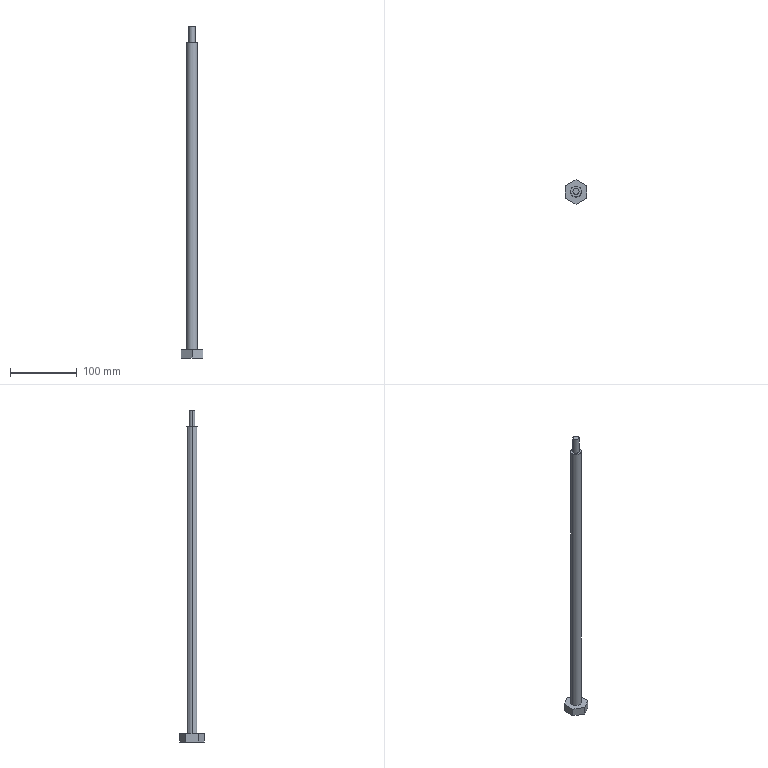Component | SolidWorks | HangerRod-1 | 1 solid | 14 faces | box 32 x 36.95 x 497 mm | volume 104721 mm3 | plane 10 | cylinder 4 | commonest cylinder face diameters 9 x2 16 x2
build123d program:
from build123d import *

# Parameters (mm, degrees)
BOSS_EXTRUDE1_DEPTH = 12
SKETCH2_R           = 8
BOSS_EXTRUDE2_DEPTH = 485
CHAMFER1_SIZE       = 1
SKETCH1_R           = 10
SKETCH1_R_2         = 4.5
CUT_EXTRUDE1_DEPTH  = 25


with BuildPart() as part:
    # Sketch1_2 → Boss-Extrude1 (new body)
    with BuildSketch(Plane.XY):
        Polygon((0, 18.475), (-16, 9.238), (-16, -9.238), (0, -18.475), (16, -9.238), (16, 9.238), align=None)
    extrude(amount=BOSS_EXTRUDE1_DEPTH)

    # Sketch2 → Boss-Extrude2 (add)
    with BuildSketch(Plane.XY.offset(12)):
        Circle(SKETCH2_R)
    extrude(amount=BOSS_EXTRUDE2_DEPTH)

    # Chamfer1
    chamfer1_edges = [part.edges().sort_by_distance(p)[0] for p in [
        (-8, 0, 497),
    ]]
    chamfer(chamfer1_edges, length=CHAMFER1_SIZE)

    # Sketch1 → Cut-Extrude1 (cut)
    with BuildSketch(Plane.XY.offset(497)):
        Circle(SKETCH1_R)
        Circle(SKETCH1_R_2, mode=Mode.SUBTRACT)
    extrude(amount=-CUT_EXTRUDE1_DEPTH, mode=Mode.SUBTRACT)


solid = part.part

# Placed as in the assembly
solid = solid.moved(Location((-917, 348, -612), (0, 0, 0)))
STEP:
#1=COLOUR_RGB('',0.7922,0.8196,0.9333);
#2=FILL_AREA_STYLE_COLOUR('',#1);
#3=FILL_AREA_STYLE('',(#2));
#4=SURFACE_STYLE_FILL_AREA(#3);
#5=SURFACE_SIDE_STYLE('',(#4));
#6=SURFACE_STYLE_USAGE(.BOTH.,#5);
#7=PRESENTATION_STYLE_ASSIGNMENT((#6));
#8=CARTESIAN_POINT('',(-35.925,13.701,-5.512));
#9=VERTEX_POINT('',#8);
#10=CARTESIAN_POINT('',(-36.28,13.701,-5.512));
#11=VERTEX_POINT('',#10);
#12=CARTESIAN_POINT('',(-36.102,13.701,-5.512));
#13=DIRECTION('',(0.,0.,1.));
#14=DIRECTION('',(1.,0.,0.));
#15=AXIS2_PLACEMENT_3D('',#12,#13,#14);
#16=CIRCLE('',#15,0.1772);
#17=EDGE_CURVE('',#9,#11,#16,.T.);
#18=ORIENTED_EDGE('',*,*,#17,.T.);
#19=CARTESIAN_POINT('',(-36.28,13.701,-4.528));
#20=VERTEX_POINT('',#19);
#21=CARTESIAN_POINT('',(-36.28,13.701,-5.512));
#22=DIRECTION('',(0.,0.,1.));
#23=VECTOR('',#22,39.37);
#24=LINE('',#21,#23);
#25=EDGE_CURVE('',#11,#20,#24,.T.);
#26=ORIENTED_EDGE('',*,*,#25,.T.);
#27=CARTESIAN_POINT('',(-35.925,13.701,-4.528));
#28=VERTEX_POINT('',#27);
#29=CARTESIAN_POINT('',(-36.102,13.701,-4.528));
#30=DIRECTION('',(0.,0.,1.));
#31=DIRECTION('',(1.,0.,0.));
#32=AXIS2_PLACEMENT_3D('',#29,#30,#31);
#33=CIRCLE('',#32,0.1772);
#34=EDGE_CURVE('',#28,#20,#33,.T.);
#35=ORIENTED_EDGE('',*,*,#34,.F.);
#36=CARTESIAN_POINT('',(-35.925,13.701,-5.512));
#37=DIRECTION('',(0.,0.,1.));
#38=VECTOR('',#37,39.37);
#39=LINE('',#36,#38);
#40=EDGE_CURVE('',#9,#28,#39,.T.);
#41=ORIENTED_EDGE('',*,*,#40,.F.);
#42=EDGE_LOOP('',(#18,#26,#35,#41));
#43=FACE_OUTER_BOUND('',#42,.T.);
#44=CARTESIAN_POINT('',(-36.102,13.701,-5.512));
#45=DIRECTION('',(0.,0.,1.));
#46=DIRECTION('',(1.,0.,0.));
#47=AXIS2_PLACEMENT_3D('',#44,#45,#46);
#48=CYLINDRICAL_SURFACE('',#47,0.1772);
#49=ADVANCED_FACE('',(#43),#48,.T.);
#50=CARTESIAN_POINT('',(-35.787,13.701,-5.512));
#51=VERTEX_POINT('',#50);
#52=CARTESIAN_POINT('',(-36.417,13.701,-5.512));
#53=VERTEX_POINT('',#52);
#54=CARTESIAN_POINT('',(-36.102,13.701,-5.512));
#55=DIRECTION('',(0.,0.,1.));
#56=DIRECTION('',(1.,0.,0.));
#57=AXIS2_PLACEMENT_3D('',#54,#55,#56);
#58=CIRCLE('',#57,0.315);
#59=EDGE_CURVE('',#51,#53,#58,.T.);
#60=ORIENTED_EDGE('',*,*,#59,.F.);
#61=CARTESIAN_POINT('',(-35.787,13.701,-23.622));
#62=VERTEX_POINT('',#61);
#63=CARTESIAN_POINT('',(-35.787,13.701,-4.528));
#64=DIRECTION('',(0.,0.,-1.));
#65=VECTOR('',#64,39.37);
#66=LINE('',#63,#65);
#67=EDGE_CURVE('',#51,#62,#66,.T.);
#68=ORIENTED_EDGE('',*,*,#67,.T.);
#69=CARTESIAN_POINT('',(-36.417,13.701,-23.622));
#70=VERTEX_POINT('',#69);
#71=CARTESIAN_POINT('',(-36.102,13.701,-23.622));
#72=DIRECTION('',(0.,0.,1.));
#73=DIRECTION('',(1.,0.,0.));
#74=AXIS2_PLACEMENT_3D('',#71,#72,#73);
#75=CIRCLE('',#74,0.315);
#76=EDGE_CURVE('',#62,#70,#75,.T.);
#77=ORIENTED_EDGE('',*,*,#76,.T.);
#78=CARTESIAN_POINT('',(-36.417,13.701,-4.528));
#79=DIRECTION('',(0.,0.,-1.));
#80=VECTOR('',#79,39.37);
#81=LINE('',#78,#80);
#82=EDGE_CURVE('',#53,#70,#81,.T.);
#83=ORIENTED_EDGE('',*,*,#82,.F.);
#84=EDGE_LOOP('',(#60,#68,#77,#83));
#85=FACE_OUTER_BOUND('',#84,.T.);
#86=CARTESIAN_POINT('',(-36.102,13.701,-4.528));
#87=DIRECTION('',(0.,0.,-1.));
#88=DIRECTION('',(-1.,0.,0.));
#89=AXIS2_PLACEMENT_3D('',#86,#87,#88);
#90=CYLINDRICAL_SURFACE('',#89,0.315);
#91=ADVANCED_FACE('',(#85),#90,.T.);
#92=ORIENTED_EDGE('',*,*,#67,.F.);
#93=CARTESIAN_POINT('',(-36.102,13.701,-5.512));
#94=DIRECTION('',(0.,0.,1.));
#95=DIRECTION('',(1.,0.,0.));
#96=AXIS2_PLACEMENT_3D('',#93,#94,#95);
#97=CIRCLE('',#96,0.315);
#98=EDGE_CURVE('',#53,#51,#97,.T.);
#99=ORIENTED_EDGE('',*,*,#98,.F.);
#100=ORIENTED_EDGE('',*,*,#82,.T.);
#101=CARTESIAN_POINT('',(-36.102,13.701,-23.622));
#102=DIRECTION('',(0.,0.,1.));
#103=DIRECTION('',(1.,0.,0.));
#104=AXIS2_PLACEMENT_3D('',#101,#102,#103);
#105=CIRCLE('',#104,0.315);
#106=EDGE_CURVE('',#70,#62,#105,.T.);
#107=ORIENTED_EDGE('',*,*,#106,.T.);
#108=EDGE_LOOP('',(#92,#99,#100,#107));
#109=FACE_OUTER_BOUND('',#108,.T.);
#110=CARTESIAN_POINT('',(-36.102,13.701,-4.528));
#111=DIRECTION('',(0.,0.,-1.));
#112=DIRECTION('',(-1.,0.,0.));
#113=AXIS2_PLACEMENT_3D('',#110,#111,#112);
#114=CYLINDRICAL_SURFACE('',#113,0.315);
#115=ADVANCED_FACE('',(#109),#114,.T.);
#116=CARTESIAN_POINT('',(-35.472,14.064,-23.622));
#117=VERTEX_POINT('',#116);
#118=CARTESIAN_POINT('',(-36.102,14.428,-23.622));
#119=VERTEX_POINT('',#118);
#120=CARTESIAN_POINT('',(-35.472,14.064,-23.622));
#121=DIRECTION('',(-0.866,0.5,0.));
#122=VECTOR('',#121,39.37);
#123=LINE('',#120,#122);
#124=EDGE_CURVE('',#117,#119,#123,.T.);
#125=ORIENTED_EDGE('',*,*,#124,.T.);
#126=CARTESIAN_POINT('',(-36.732,14.064,-23.622));
#127=VERTEX_POINT('',#126);
#128=CARTESIAN_POINT('',(-36.102,14.428,-23.622));
#129=DIRECTION('',(-0.866,-0.5,0.));
#130=VECTOR('',#129,39.37);
#131=LINE('',#128,#130);
#132=EDGE_CURVE('',#119,#127,#131,.T.);
#133=ORIENTED_EDGE('',*,*,#132,.T.);
#134=CARTESIAN_POINT('',(-36.732,13.337,-23.622));
#135=VERTEX_POINT('',#134);
#136=CARTESIAN_POINT('',(-36.732,14.064,-23.622));
#137=DIRECTION('',(0.,-1.,0.));
#138=VECTOR('',#137,39.37);
#139=LINE('',#136,#138);
#140=EDGE_CURVE('',#127,#135,#139,.T.);
#141=ORIENTED_EDGE('',*,*,#140,.T.);
#142=CARTESIAN_POINT('',(-36.102,12.973,-23.622));
#143=VERTEX_POINT('',#142);
#144=CARTESIAN_POINT('',(-36.732,13.337,-23.622));
#145=DIRECTION('',(0.866,-0.5,0.));
#146=VECTOR('',#145,39.37);
#147=LINE('',#144,#146);
#148=EDGE_CURVE('',#135,#143,#147,.T.);
#149=ORIENTED_EDGE('',*,*,#148,.T.);
#150=CARTESIAN_POINT('',(-35.472,13.337,-23.622));
#151=VERTEX_POINT('',#150);
#152=CARTESIAN_POINT('',(-36.102,12.973,-23.622));
#153=DIRECTION('',(0.866,0.5,0.));
#154=VECTOR('',#153,39.37);
#155=LINE('',#152,#154);
#156=EDGE_CURVE('',#143,#151,#155,.T.);
#157=ORIENTED_EDGE('',*,*,#156,.T.);
#158=CARTESIAN_POINT('',(-35.472,13.337,-23.622));
#159=DIRECTION('',(-0.,1.,0.));
#160=VECTOR('',#159,39.37);
#161=LINE('',#158,#160);
#162=EDGE_CURVE('',#151,#117,#161,.T.);
#163=ORIENTED_EDGE('',*,*,#162,.T.);
#164=EDGE_LOOP('',(#125,#133,#141,#149,#157,#163));
#165=FACE_OUTER_BOUND('',#164,.T.);
#166=ORIENTED_EDGE('',*,*,#106,.F.);
#167=ORIENTED_EDGE('',*,*,#76,.F.);
#168=EDGE_LOOP('',(#166,#167));
#169=FACE_BOUND('',#168,.T.);
#170=CARTESIAN_POINT('',(-36.102,13.701,-23.622));
#171=DIRECTION('',(0.,0.,1.));
#172=DIRECTION('',(1.,0.,0.));
#173=AXIS2_PLACEMENT_3D('',#170,#171,#172);
#174=PLANE('',#173);
#175=ADVANCED_FACE('',(#165,#169),#174,.T.);
#176=CARTESIAN_POINT('',(-35.472,14.064,-24.094));
#177=VERTEX_POINT('',#176);
#178=CARTESIAN_POINT('',(-36.102,14.428,-24.094));
#179=VERTEX_POINT('',#178);
#180=CARTESIAN_POINT('',(-35.472,14.064,-24.094));
#181=DIRECTION('',(-0.866,0.5,0.));
#182=VECTOR('',#181,39.37);
#183=LINE('',#180,#182);
#184=EDGE_CURVE('',#177,#179,#183,.T.);
#185=ORIENTED_EDGE('',*,*,#184,.T.);
#186=CARTESIAN_POINT('',(-36.102,14.428,-23.622));
#187=DIRECTION('',(0.,0.,-1.));
#188=VECTOR('',#187,39.37);
#189=LINE('',#186,#188);
#190=EDGE_CURVE('',#119,#179,#189,.T.);
#191=ORIENTED_EDGE('',*,*,#190,.F.);
#192=ORIENTED_EDGE('',*,*,#124,.F.);
#193=CARTESIAN_POINT('',(-35.472,14.064,-23.622));
#194=DIRECTION('',(0.,0.,-1.));
#195=VECTOR('',#194,39.37);
#196=LINE('',#193,#195);
#197=EDGE_CURVE('',#117,#177,#196,.T.);
#198=ORIENTED_EDGE('',*,*,#197,.T.);
#199=EDGE_LOOP('',(#185,#191,#192,#198));
#200=FACE_OUTER_BOUND('',#199,.T.);
#201=CARTESIAN_POINT('',(-35.472,14.064,-23.622));
#202=DIRECTION('',(-0.5,-0.866,0.));
#203=DIRECTION('',(0.866,-0.5,0.));
#204=AXIS2_PLACEMENT_3D('',#201,#202,#203);
#205=PLANE('',#204);
#206=ADVANCED_FACE('',(#200),#205,.F.);
#207=CARTESIAN_POINT('',(-36.732,14.064,-24.094));
#208=VERTEX_POINT('',#207);
#209=CARTESIAN_POINT('',(-36.102,14.428,-24.094));
#210=DIRECTION('',(-0.866,-0.5,0.));
#211=VECTOR('',#210,39.37);
#212=LINE('',#209,#211);
#213=EDGE_CURVE('',#179,#208,#212,.T.);
#214=ORIENTED_EDGE('',*,*,#213,.T.);
#215=CARTESIAN_POINT('',(-36.732,14.064,-23.622));
#216=DIRECTION('',(0.,0.,-1.));
#217=VECTOR('',#216,39.37);
#218=LINE('',#215,#217);
#219=EDGE_CURVE('',#127,#208,#218,.T.);
#220=ORIENTED_EDGE('',*,*,#219,.F.);
#221=ORIENTED_EDGE('',*,*,#132,.F.);
#222=ORIENTED_EDGE('',*,*,#190,.T.);
#223=EDGE_LOOP('',(#214,#220,#221,#222));
#224=FACE_OUTER_BOUND('',#223,.T.);
#225=CARTESIAN_POINT('',(-36.102,14.428,-23.622));
#226=DIRECTION('',(0.5,-0.866,0.));
#227=DIRECTION('',(0.866,0.5,0.));
#228=AXIS2_PLACEMENT_3D('',#225,#226,#227);
#229=PLANE('',#228);
#230=ADVANCED_FACE('',(#224),#229,.F.);
#231=CARTESIAN_POINT('',(-36.732,13.337,-24.094));
#232=VERTEX_POINT('',#231);
#233=CARTESIAN_POINT('',(-36.732,14.064,-24.094));
#234=DIRECTION('',(0.,-1.,0.));
#235=VECTOR('',#234,39.37);
#236=LINE('',#233,#235);
#237=EDGE_CURVE('',#208,#232,#236,.T.);
#238=ORIENTED_EDGE('',*,*,#237,.T.);
#239=CARTESIAN_POINT('',(-36.732,13.337,-23.622));
#240=DIRECTION('',(0.,0.,-1.));
#241=VECTOR('',#240,39.37);
#242=LINE('',#239,#241);
#243=EDGE_CURVE('',#135,#232,#242,.T.);
#244=ORIENTED_EDGE('',*,*,#243,.F.);
#245=ORIENTED_EDGE('',*,*,#140,.F.);
#246=ORIENTED_EDGE('',*,*,#219,.T.);
#247=EDGE_LOOP('',(#238,#244,#245,#246));
#248=FACE_OUTER_BOUND('',#247,.T.);
#249=CARTESIAN_POINT('',(-36.732,14.064,-23.622));
#250=DIRECTION('',(1.,0.,0.));
#251=DIRECTION('',(-0.,1.,0.));
#252=AXIS2_PLACEMENT_3D('',#249,#250,#251);
#253=PLANE('',#252);
#254=ADVANCED_FACE('',(#248),#253,.F.);
#255=CARTESIAN_POINT('',(-36.102,12.973,-24.094));
#256=VERTEX_POINT('',#255);
#257=CARTESIAN_POINT('',(-36.732,13.337,-24.094));
#258=DIRECTION('',(0.866,-0.5,0.));
#259=VECTOR('',#258,39.37);
#260=LINE('',#257,#259);
#261=EDGE_CURVE('',#232,#256,#260,.T.);
#262=ORIENTED_EDGE('',*,*,#261,.T.);
#263=CARTESIAN_POINT('',(-36.102,12.973,-23.622));
#264=DIRECTION('',(0.,0.,-1.));
#265=VECTOR('',#264,39.37);
#266=LINE('',#263,#265);
#267=EDGE_CURVE('',#143,#256,#266,.T.);
#268=ORIENTED_EDGE('',*,*,#267,.F.);
#269=ORIENTED_EDGE('',*,*,#148,.F.);
#270=ORIENTED_EDGE('',*,*,#243,.T.);
#271=EDGE_LOOP('',(#262,#268,#269,#270));
#272=FACE_OUTER_BOUND('',#271,.T.);
#273=CARTESIAN_POINT('',(-36.732,13.337,-23.622));
#274=DIRECTION('',(0.5,0.866,0.));
#275=DIRECTION('',(-0.866,0.5,0.));
#276=AXIS2_PLACEMENT_3D('',#273,#274,#275);
#277=PLANE('',#276);
#278=ADVANCED_FACE('',(#272),#277,.F.);
#279=CARTESIAN_POINT('',(-35.472,13.337,-24.094));
#280=VERTEX_POINT('',#279);
#281=CARTESIAN_POINT('',(-36.102,12.973,-24.094));
#282=DIRECTION('',(0.866,0.5,0.));
#283=VECTOR('',#282,39.37);
#284=LINE('',#281,#283);
#285=EDGE_CURVE('',#256,#280,#284,.T.);
#286=ORIENTED_EDGE('',*,*,#285,.T.);
#287=CARTESIAN_POINT('',(-35.472,13.337,-23.622));
#288=DIRECTION('',(0.,0.,-1.));
#289=VECTOR('',#288,39.37);
#290=LINE('',#287,#289);
#291=EDGE_CURVE('',#151,#280,#290,.T.);
#292=ORIENTED_EDGE('',*,*,#291,.F.);
#293=ORIENTED_EDGE('',*,*,#156,.F.);
#294=ORIENTED_EDGE('',*,*,#267,.T.);
#295=EDGE_LOOP('',(#286,#292,#293,#294));
#296=FACE_OUTER_BOUND('',#295,.T.);
#297=CARTESIAN_POINT('',(-36.102,12.973,-23.622));
#298=DIRECTION('',(-0.5,0.866,0.));
#299=DIRECTION('',(-0.866,-0.5,0.));
#300=AXIS2_PLACEMENT_3D('',#297,#298,#299);
#301=PLANE('',#300);
#302=ADVANCED_FACE('',(#296),#301,.F.);
#303=CARTESIAN_POINT('',(-35.472,13.337,-24.094));
#304=DIRECTION('',(-0.,1.,0.));
#305=VECTOR('',#304,39.37);
#306=LINE('',#303,#305);
#307=EDGE_CURVE('',#280,#177,#306,.T.);
#308=ORIENTED_EDGE('',*,*,#307,.T.);
#309=ORIENTED_EDGE('',*,*,#197,.F.);
#310=ORIENTED_EDGE('',*,*,#162,.F.);
#311=ORIENTED_EDGE('',*,*,#291,.T.);
#312=EDGE_LOOP('',(#308,#309,#310,#311));
#313=FACE_OUTER_BOUND('',#312,.T.);
#314=CARTESIAN_POINT('',(-35.472,13.337,-23.622));
#315=DIRECTION('',(-1.,-0.,0.));
#316=DIRECTION('',(0.,-1.,0.));
#317=AXIS2_PLACEMENT_3D('',#314,#315,#316);
#318=PLANE('',#317);
#319=ADVANCED_FACE('',(#313),#318,.F.);
#320=ORIENTED_EDGE('',*,*,#184,.F.);
#321=ORIENTED_EDGE('',*,*,#307,.F.);
#322=ORIENTED_EDGE('',*,*,#285,.F.);
#323=ORIENTED_EDGE('',*,*,#261,.F.);
#324=ORIENTED_EDGE('',*,*,#237,.F.);
#325=ORIENTED_EDGE('',*,*,#213,.F.);
#326=EDGE_LOOP('',(#320,#321,#322,#323,#324,#325));
#327=FACE_OUTER_BOUND('',#326,.T.);
#328=CARTESIAN_POINT('',(-36.102,13.701,-24.094));
#329=DIRECTION('',(0.,0.,1.));
#330=DIRECTION('',(1.,0.,0.));
#331=AXIS2_PLACEMENT_3D('',#328,#329,#330);
#332=PLANE('',#331);
#333=ADVANCED_FACE('',(#327),#332,.F.);
#334=ORIENTED_EDGE('',*,*,#17,.F.);
#335=CARTESIAN_POINT('',(-36.102,13.701,-5.512));
#336=DIRECTION('',(0.,0.,1.));
#337=DIRECTION('',(1.,0.,0.));
#338=AXIS2_PLACEMENT_3D('',#335,#336,#337);
#339=CIRCLE('',#338,0.1772);
#340=EDGE_CURVE('',#11,#9,#339,.T.);
#341=ORIENTED_EDGE('',*,*,#340,.F.);
#342=EDGE_LOOP('',(#334,#341));
#343=FACE_BOUND('',#342,.T.);
#344=ORIENTED_EDGE('',*,*,#98,.T.);
#345=ORIENTED_EDGE('',*,*,#59,.T.);
#346=EDGE_LOOP('',(#344,#345));
#347=FACE_OUTER_BOUND('',#346,.T.);
#348=CARTESIAN_POINT('',(-36.102,13.701,-5.512));
#349=DIRECTION('',(0.,0.,1.));
#350=DIRECTION('',(1.,0.,0.));
#351=AXIS2_PLACEMENT_3D('',#348,#349,#350);
#352=PLANE('',#351);
#353=ADVANCED_FACE('',(#343,#347),#352,.T.);
#354=ORIENTED_EDGE('',*,*,#25,.F.);
#355=ORIENTED_EDGE('',*,*,#340,.T.);
#356=ORIENTED_EDGE('',*,*,#40,.T.);
#357=CARTESIAN_POINT('',(-36.102,13.701,-4.528));
#358=DIRECTION('',(0.,0.,1.));
#359=DIRECTION('',(1.,0.,0.));
#360=AXIS2_PLACEMENT_3D('',#357,#358,#359);
#361=CIRCLE('',#360,0.1772);
#362=EDGE_CURVE('',#20,#28,#361,.T.);
#363=ORIENTED_EDGE('',*,*,#362,.F.);
#364=EDGE_LOOP('',(#354,#355,#356,#363));
#365=FACE_OUTER_BOUND('',#364,.T.);
#366=CARTESIAN_POINT('',(-36.102,13.701,-5.512));
#367=DIRECTION('',(0.,0.,1.));
#368=DIRECTION('',(1.,0.,0.));
#369=AXIS2_PLACEMENT_3D('',#366,#367,#368);
#370=CYLINDRICAL_SURFACE('',#369,0.1772);
#371=ADVANCED_FACE('',(#365),#370,.T.);
#372=ORIENTED_EDGE('',*,*,#34,.T.);
#373=ORIENTED_EDGE('',*,*,#362,.T.);
#374=EDGE_LOOP('',(#372,#373));
#375=FACE_OUTER_BOUND('',#374,.T.);
#376=CARTESIAN_POINT('',(-36.102,13.701,-4.528));
#377=DIRECTION('',(0.,0.,1.));
#378=DIRECTION('',(1.,0.,0.));
#379=AXIS2_PLACEMENT_3D('',#376,#377,#378);
#380=PLANE('',#379);
#381=ADVANCED_FACE('',(#375),#380,.T.);
#382=CLOSED_SHELL('',(#49,#91,#115,#175,#206,#230,#254,#278,#302,#319,#333,#353,#371,#381));
#383=MANIFOLD_SOLID_BREP('',#382);
#384=STYLED_ITEM('',(#7),#383);
#385=(LENGTH_UNIT()NAMED_UNIT(*)SI_UNIT($,.METRE.));
#386=LENGTH_MEASURE_WITH_UNIT(LENGTH_MEASURE(0.0254),#385);
#387=DIMENSIONAL_EXPONENTS(1.,0.,0.,0.,0.,0.,0.);
#388=(CONVERSION_BASED_UNIT('',#386)LENGTH_UNIT()NAMED_UNIT(#387));
#389=UNCERTAINTY_MEASURE_WITH_UNIT(LENGTH_MEASURE(0.00001),#388,'','');
#390=(NAMED_UNIT(*)PLANE_ANGLE_UNIT()SI_UNIT($,.RADIAN.));
#391=(NAMED_UNIT(*)SI_UNIT($,.STERADIAN.)SOLID_ANGLE_UNIT());
#392=(GEOMETRIC_REPRESENTATION_CONTEXT(3)GLOBAL_UNCERTAINTY_ASSIGNED_CONTEXT((#389))GLOBAL_UNIT_ASSIGNED_CONTEXT((#388,#390,#391))REPRESENTATION_CONTEXT('',''));
#393=MECHANICAL_DESIGN_GEOMETRIC_PRESENTATION_REPRESENTATION('',(#384),#392);
#394=CARTESIAN_POINT('',(0.,0.,0.));
#395=DIRECTION('',(0.,0.,1.));
#396=DIRECTION('',(1.,0.,0.));
#397=AXIS2_PLACEMENT_3D('',#394,#395,#396);
#398=(LENGTH_UNIT()NAMED_UNIT(*)SI_UNIT($,.METRE.));
#399=LENGTH_MEASURE_WITH_UNIT(LENGTH_MEASURE(0.0254),#398);
#400=DIMENSIONAL_EXPONENTS(1.,0.,0.,0.,0.,0.,0.);
#401=(CONVERSION_BASED_UNIT('',#399)LENGTH_UNIT()NAMED_UNIT(#400));
#402=UNCERTAINTY_MEASURE_WITH_UNIT(LENGTH_MEASURE(0.00001),#401,'','');
#403=(NAMED_UNIT(*)PLANE_ANGLE_UNIT()SI_UNIT($,.RADIAN.));
#404=(NAMED_UNIT(*)SI_UNIT($,.STERADIAN.)SOLID_ANGLE_UNIT());
#405=(GEOMETRIC_REPRESENTATION_CONTEXT(3)GLOBAL_UNCERTAINTY_ASSIGNED_CONTEXT((#402))GLOBAL_UNIT_ASSIGNED_CONTEXT((#401,#403,#404))REPRESENTATION_CONTEXT('',''));
#406=ADVANCED_BREP_SHAPE_REPRESENTATION('',(#383,#397),#405);
#407=PRESENTATION_LAYER_ASSIGNMENT('','',(#384));